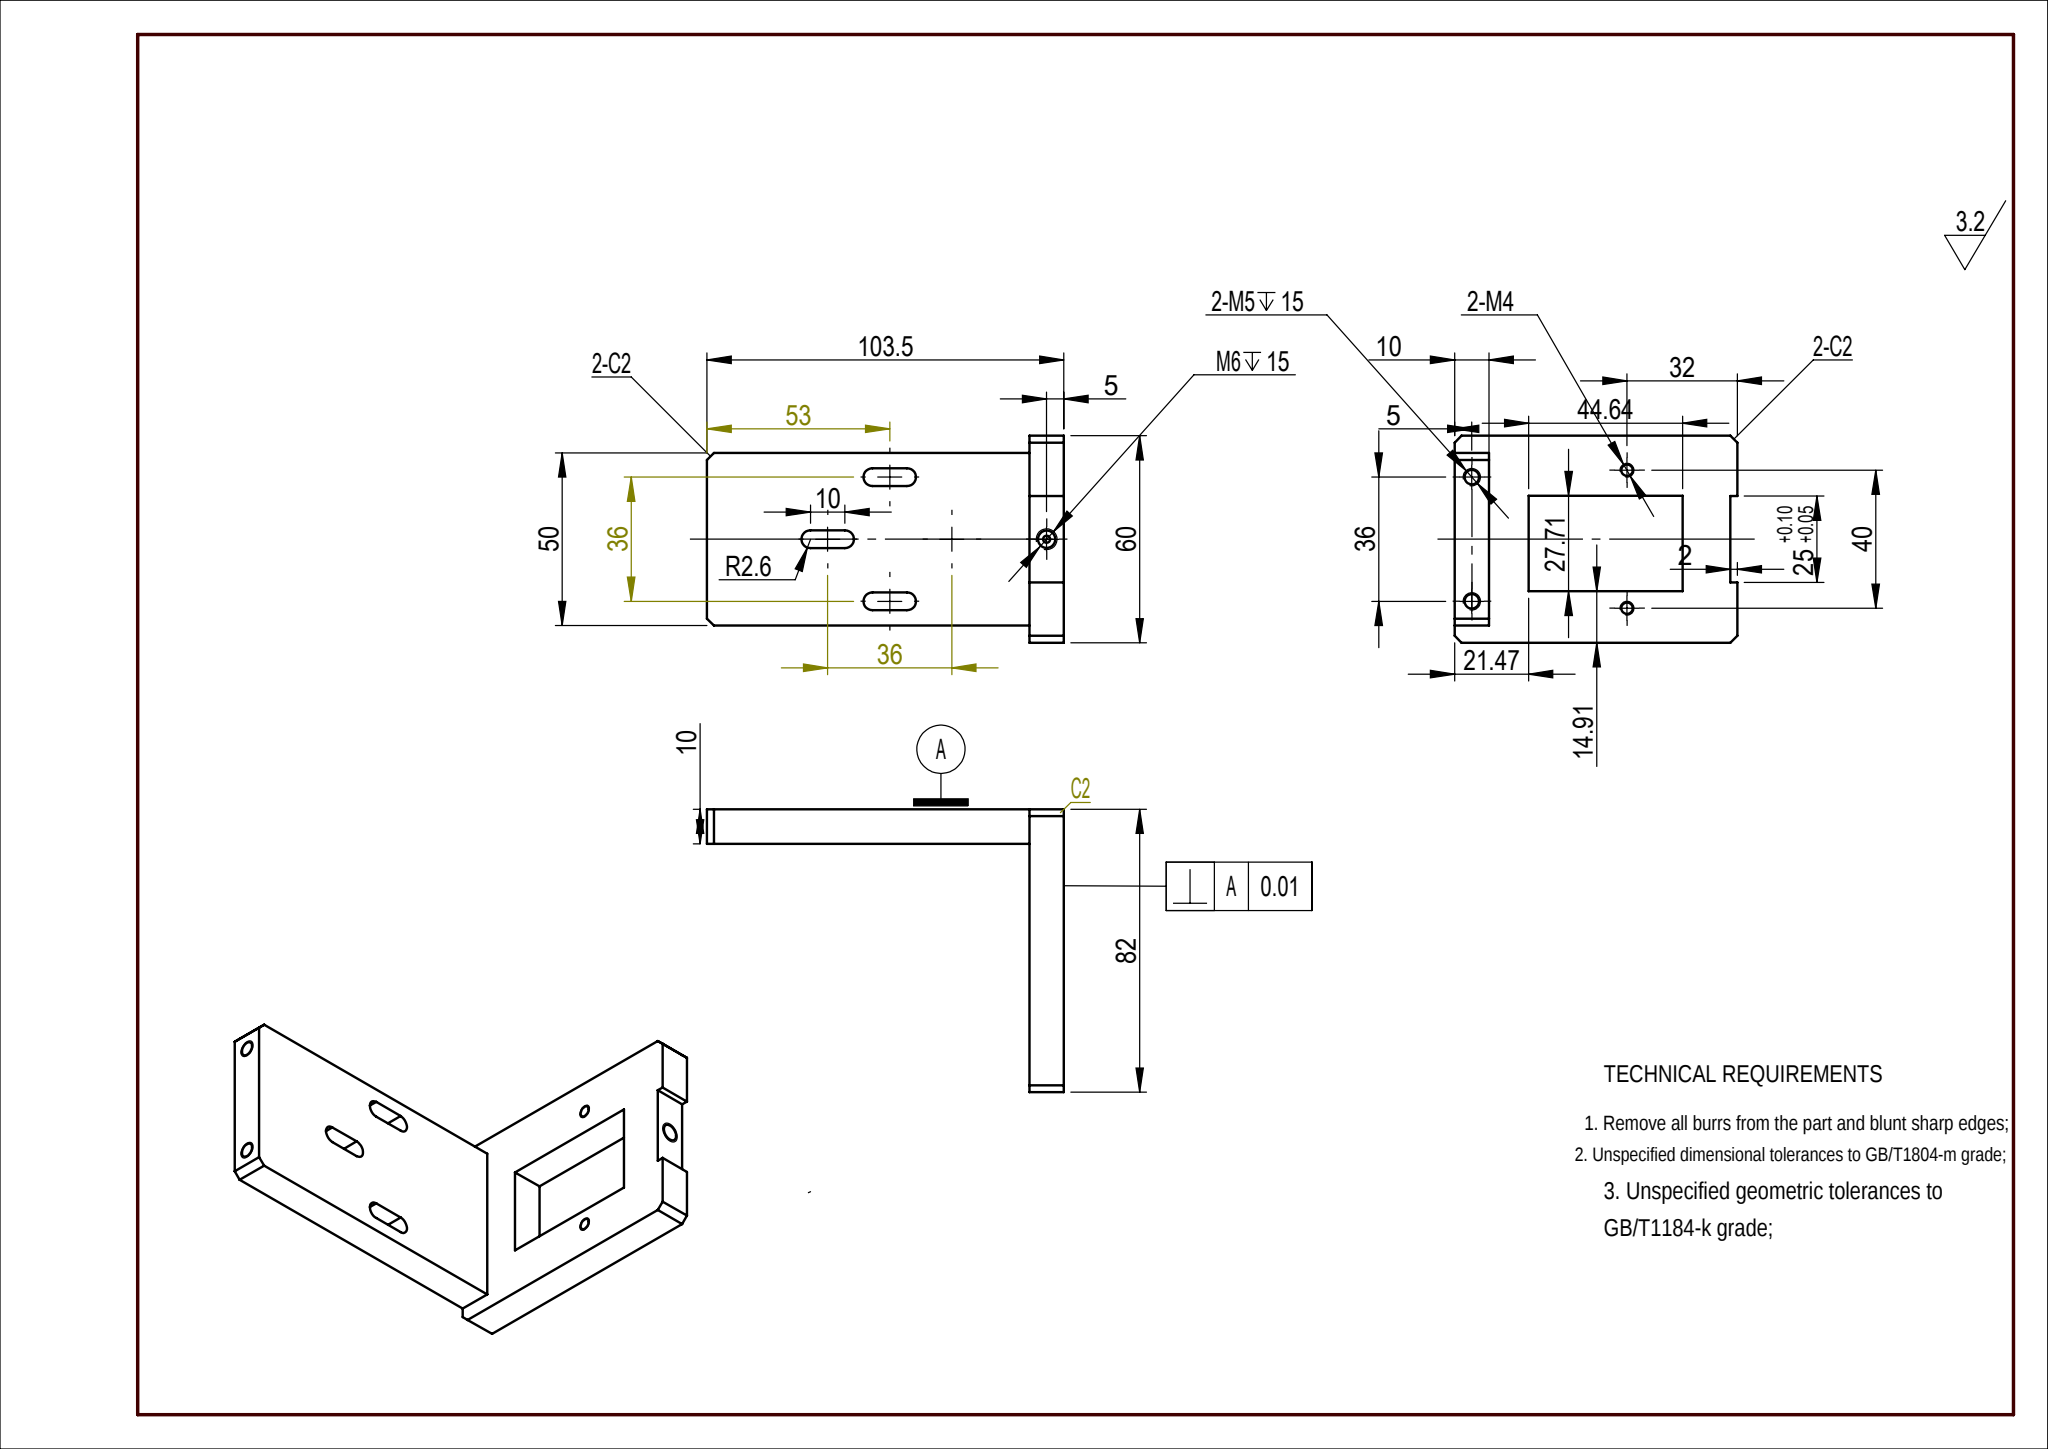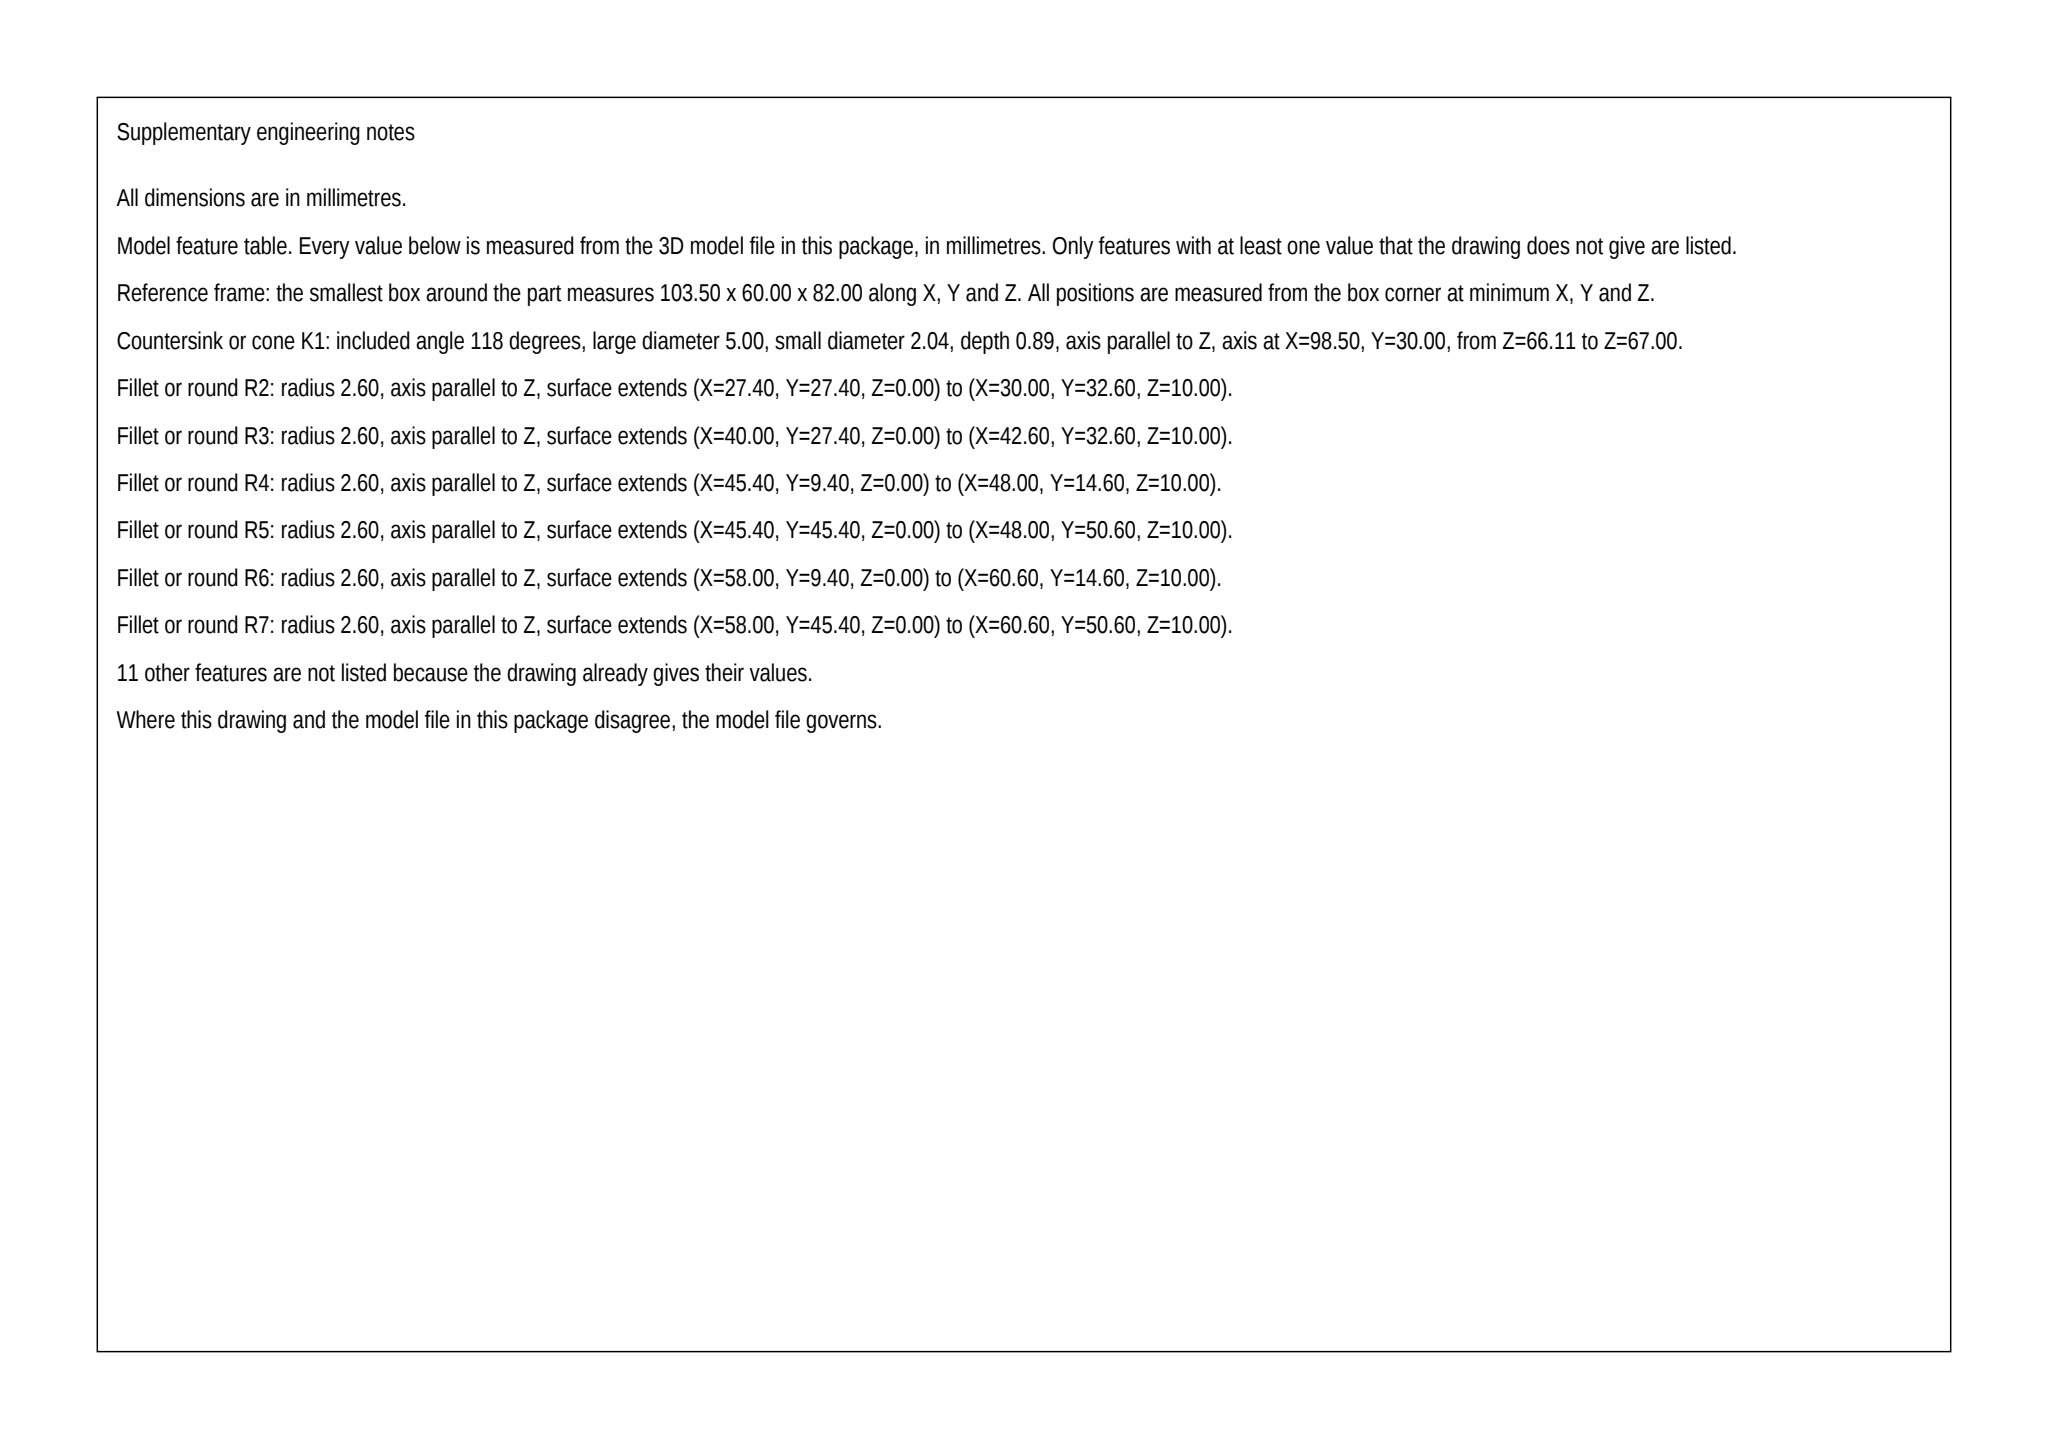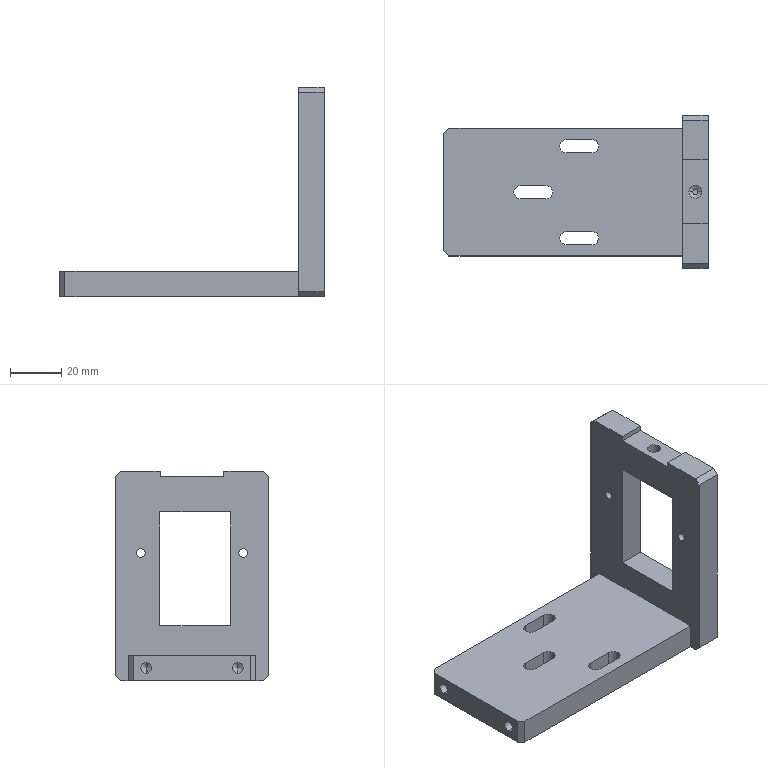Part | SolidWorks | mm | 1 solid | 55 faces | box 103.5 x 60 x 82 mm | volume 79808 mm3 | plane 30 | cylinder 19 | cone 6 | commonest cylinder face diameters 5.2 x9 3.3 x4 4.2 x4 5 x2
build123d program:
from build123d import *

# Parameters (mm, degrees)
SKETCH1_W                = 102
SKETCH1_H                = 50
BOSS_EXTRUDE1_DEPTH      = 5
M5_TAPPED_HOLE1_D        = 4.2
M5_TAPPED_HOLE1_DEPTH    = 18.4
M5_TAPPED_HOLE1_TIP      = 1.262
BOSS_EXTRUDE2_DEPTH      = 72
BOSS_EXTRUDE2_DEPTH_BACK = 10
SKETCH11_W               = 10
SKETCH11_H               = 60
M4_TAPPED_HOLE1_D        = 3.3
M6_TAPPED_HOLE1_D        = 5
M6_TAPPED_HOLE1_DEPTH    = 15
M6_TAPPED_HOLE1_TIP      = 1.502
CHAMFER1_SIZE            = 2
SKETCH21_W               = 2
SKETCH21_H               = 25
CUT_EXTRUDE1_DEPTH       = 154.898
CUT_EXTRUDE2_DEPTH       = 95.023
SKETCH23_W               = 44.641
SKETCH23_H               = 27.706
CUT_EXTRUDE3_DEPTH       = 22


with BuildPart() as part:
    # Sketch1 → Boss-Extrude1 (new, symmetric)
    with BuildSketch(Plane.XY):
        Rectangle(SKETCH1_W, SKETCH1_H)
    extrude(amount=BOSS_EXTRUDE1_DEPTH, both=True)

    # M5 Tapped Hole1
    with Locations(Plane(origin=(-51, 16.003, -1.338), x_dir=(0, 0, -1), z_dir=(-1, 0, 0))):
        with Locations((-1.338, -1.997), (-1.338, 34.003)):
            Hole(M5_TAPPED_HOLE1_D / 2, depth=M5_TAPPED_HOLE1_DEPTH)
            with Locations((0, 0, -(M5_TAPPED_HOLE1_DEPTH + M5_TAPPED_HOLE1_TIP / 2))):  # 118° drill point
                Cone(0, M5_TAPPED_HOLE1_D / 2, M5_TAPPED_HOLE1_TIP, mode=Mode.SUBTRACT)

    # Sketch11 → Boss-Extrude2 (add, two sides: drawn at the far end of the back side and taken through both)
    with BuildSketch(Plane.XY.offset(5).offset(-BOSS_EXTRUDE2_DEPTH_BACK)):
        with Locations((47.5, 0)):
            Rectangle(SKETCH11_W, SKETCH11_H)
    extrude(amount=BOSS_EXTRUDE2_DEPTH + BOSS_EXTRUDE2_DEPTH_BACK)

    # M4 Tapped Hole1 (through all)
    with Locations(Plane.ZY.offset(-42.5)):
        with Locations((45, 20), (45, -20)):
            Hole(M4_TAPPED_HOLE1_D / 2)

    # M6 Tapped Hole1
    with Locations(Plane.XY.offset(77)):
        with Locations((47.5, 0)):
            Hole(M6_TAPPED_HOLE1_D / 2, depth=M6_TAPPED_HOLE1_DEPTH)
            with Locations((0, 0, -(M6_TAPPED_HOLE1_DEPTH + M6_TAPPED_HOLE1_TIP / 2))):  # 118° drill point
                Cone(0, M6_TAPPED_HOLE1_D / 2, M6_TAPPED_HOLE1_TIP, mode=Mode.SUBTRACT)

    # Chamfer1
    chamfer1_edges = [part.edges().sort_by_distance(p)[0] for p in [
        (47.5, -30, -5),
        (47.5, 30, -5),
        (47.5, 30, 77),
        (47.5, -30, 77),
        (-51, -25, 0),
        (-51, 25, 0),
    ]]
    chamfer(chamfer1_edges, length=CHAMFER1_SIZE)

    # Sketch21 → Cut-Extrude1 (cut, through all)
    with BuildSketch(Plane(origin=(42.5, 0, 113.5), x_dir=(0, 0, -1), z_dir=(1, 0, 0))):
        with Locations((37.5, 0)):
            Rectangle(SKETCH21_W, SKETCH21_H)
    extrude(amount=CUT_EXTRUDE1_DEPTH, mode=Mode.SUBTRACT)

    # Sketch22 → Cut-Extrude2 (cut, through all)
    with BuildSketch(Plane.XY.offset(5)):
        with BuildLine():
            Line((-11, -2.6), (-21, -2.6))
            ThreePointArc((-21, -2.6), (-23.6, 0), (-21, 2.6))
            Line((-21, 2.6), (-11, 2.6))
            ThreePointArc((-11, 2.6), (-8.4, 0), (-11, -2.6))
        make_face()
        with BuildLine():
            Line((-3, -15.4), (7, -15.4))
            ThreePointArc((7, -15.4), (9.6, -18), (7, -20.6))
            Line((7, -20.6), (-3, -20.6))
            ThreePointArc((-3, -20.6), (-5.6, -18), (-3, -15.4))
        make_face()
        with BuildLine():
            Line((-3, 15.4), (7, 15.4))
            ThreePointArc((7, 15.4), (9.6, 18), (7, 20.6))
            Line((7, 20.6), (-3, 20.6))
            ThreePointArc((-3, 20.6), (-5.6, 18), (-3, 15.4))
        make_face()
    extrude(amount=-CUT_EXTRUDE2_DEPTH, mode=Mode.SUBTRACT)

    # Sketch23 → Cut-Extrude3 (cut)
    with BuildSketch(Plane.ZY.offset(-42.5)):
        with Locations((38.79, -1.233)):
            Rectangle(SKETCH23_W, SKETCH23_H)
    extrude(amount=-CUT_EXTRUDE3_DEPTH, mode=Mode.SUBTRACT)


solid = part.part